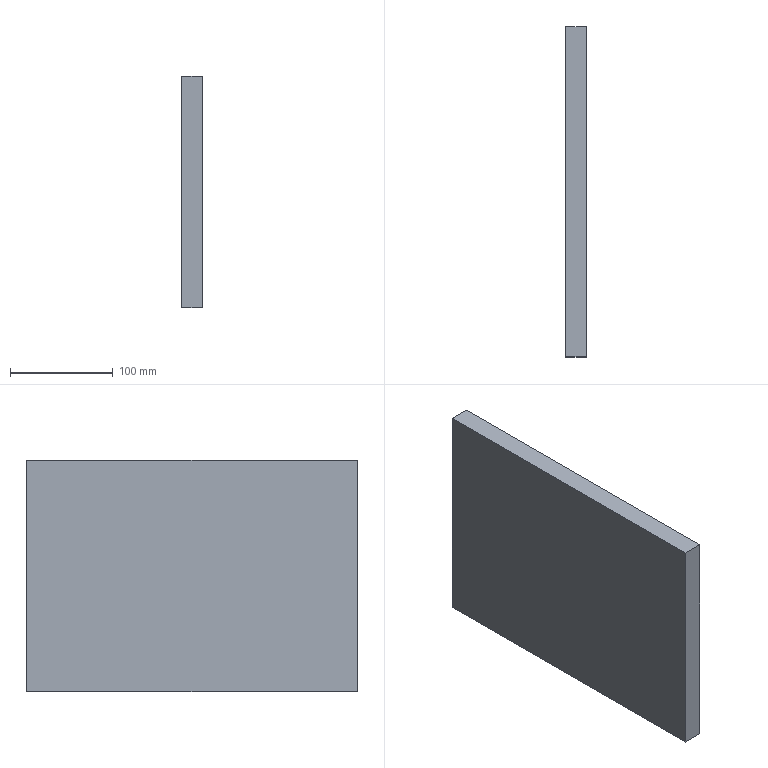Component | NX | CH3404_5-3 | 1 solid | 6 faces | box 20 x 321 x 225 mm | volume 1444500 mm3 | plane 6
STEP:
#1=CARTESIAN_POINT('',(0.,0.,0.));
#2=DIRECTION('',(0.,0.,1.));
#3=DIRECTION('',(1.,0.,0.));
#4=AXIS2_PLACEMENT_3D('',#1,#2,#3);
#5=CARTESIAN_POINT('',(115.,-160.5,0.));
#6=VERTEX_POINT('',#5);
#7=CARTESIAN_POINT('',(115.,160.5,-0.));
#8=VERTEX_POINT('',#7);
#9=CARTESIAN_POINT('',(115.,-160.5,0.));
#10=DIRECTION('',(0.,1.,-0.));
#11=VECTOR('',#10,1.);
#12=LINE('',#9,#11);
#13=CARTESIAN_POINT('',(95.,-160.5,0.));
#14=DIRECTION('',(0.,-0.,-1.));
#15=DIRECTION('',(0.,-1.,0.));
#16=AXIS2_PLACEMENT_3D('',#13,#14,#15);
#17=PLANE('',#16);
#18=CARTESIAN_POINT('',(0.,-20.));
#19=DIRECTION('',(-1.,0.));
#20=VECTOR('',#19,1.);
#21=LINE('',#18,#20);
#22=(GEOMETRIC_REPRESENTATION_CONTEXT(2)PARAMETRIC_REPRESENTATION_CONTEXT()REPRESENTATION_CONTEXT('',''));
#23=DEFINITIONAL_REPRESENTATION('',(#21),#22);
#24=PCURVE('',#17,#23);
#25=CARTESIAN_POINT('',(115.,160.5,-112.5));
#26=DIRECTION('',(-1.,0.,0.));
#27=DIRECTION('',(0.,1.,0.));
#28=AXIS2_PLACEMENT_3D('',#25,#26,#27);
#29=PLANE('',#28);
#30=CARTESIAN_POINT('',(-321.,-112.5));
#31=DIRECTION('',(1.,0.));
#32=VECTOR('',#31,1.);
#33=LINE('',#30,#32);
#34=(GEOMETRIC_REPRESENTATION_CONTEXT(2)PARAMETRIC_REPRESENTATION_CONTEXT()REPRESENTATION_CONTEXT('',''));
#35=DEFINITIONAL_REPRESENTATION('',(#33),#34);
#36=PCURVE('',#29,#35);
#37=SURFACE_CURVE('',#12,(#24,#36),.PCURVE_S1.);
#38=EDGE_CURVE('',#6,#8,#37,.T.);
#39=ORIENTED_EDGE('',*,*,#38,.T.);
#40=CARTESIAN_POINT('',(95.,160.5,-0.));
#41=VERTEX_POINT('',#40);
#42=CARTESIAN_POINT('',(95.,160.5,-0.));
#43=DIRECTION('',(1.,0.,0.));
#44=VECTOR('',#43,1.);
#45=LINE('',#42,#44);
#46=CARTESIAN_POINT('',(-321.,0.));
#47=DIRECTION('',(0.,-1.));
#48=VECTOR('',#47,1.);
#49=LINE('',#46,#48);
#50=(GEOMETRIC_REPRESENTATION_CONTEXT(2)PARAMETRIC_REPRESENTATION_CONTEXT()REPRESENTATION_CONTEXT('',''));
#51=DEFINITIONAL_REPRESENTATION('',(#49),#50);
#52=PCURVE('',#17,#51);
#53=CARTESIAN_POINT('',(95.,160.5,-0.));
#54=DIRECTION('',(0.,-1.,0.));
#55=DIRECTION('',(-1.,0.,0.));
#56=AXIS2_PLACEMENT_3D('',#53,#54,#55);
#57=PLANE('',#56);
#58=CARTESIAN_POINT('',(0.,0.));
#59=DIRECTION('',(-1.,0.));
#60=VECTOR('',#59,1.);
#61=LINE('',#58,#60);
#62=(GEOMETRIC_REPRESENTATION_CONTEXT(2)PARAMETRIC_REPRESENTATION_CONTEXT()REPRESENTATION_CONTEXT('',''));
#63=DEFINITIONAL_REPRESENTATION('',(#61),#62);
#64=PCURVE('',#57,#63);
#65=SURFACE_CURVE('',#45,(#52,#64),.PCURVE_S1.);
#66=EDGE_CURVE('',#41,#8,#65,.T.);
#67=ORIENTED_EDGE('',*,*,#66,.F.);
#68=CARTESIAN_POINT('',(95.,-160.5,0.));
#69=VERTEX_POINT('',#68);
#70=CARTESIAN_POINT('',(95.,-160.5,0.));
#71=DIRECTION('',(0.,1.,-0.));
#72=VECTOR('',#71,1.);
#73=LINE('',#70,#72);
#74=CARTESIAN_POINT('',(0.,0.));
#75=DIRECTION('',(-1.,0.));
#76=VECTOR('',#75,1.);
#77=LINE('',#74,#76);
#78=(GEOMETRIC_REPRESENTATION_CONTEXT(2)PARAMETRIC_REPRESENTATION_CONTEXT()REPRESENTATION_CONTEXT('',''));
#79=DEFINITIONAL_REPRESENTATION('',(#77),#78);
#80=PCURVE('',#17,#79);
#81=CARTESIAN_POINT('',(95.,160.5,-112.5));
#82=DIRECTION('',(-1.,0.,0.));
#83=DIRECTION('',(0.,1.,0.));
#84=AXIS2_PLACEMENT_3D('',#81,#82,#83);
#85=PLANE('',#84);
#86=CARTESIAN_POINT('',(-321.,-112.5));
#87=DIRECTION('',(1.,0.));
#88=VECTOR('',#87,1.);
#89=LINE('',#86,#88);
#90=(GEOMETRIC_REPRESENTATION_CONTEXT(2)PARAMETRIC_REPRESENTATION_CONTEXT()REPRESENTATION_CONTEXT('',''));
#91=DEFINITIONAL_REPRESENTATION('',(#89),#90);
#92=PCURVE('',#85,#91);
#93=SURFACE_CURVE('',#73,(#80,#92),.PCURVE_S1.);
#94=EDGE_CURVE('',#69,#41,#93,.T.);
#95=ORIENTED_EDGE('',*,*,#94,.F.);
#96=CARTESIAN_POINT('',(95.,-160.5,0.));
#97=DIRECTION('',(1.,0.,0.));
#98=VECTOR('',#97,1.);
#99=LINE('',#96,#98);
#100=CARTESIAN_POINT('',(0.,0.));
#101=DIRECTION('',(0.,-1.));
#102=VECTOR('',#101,1.);
#103=LINE('',#100,#102);
#104=(GEOMETRIC_REPRESENTATION_CONTEXT(2)PARAMETRIC_REPRESENTATION_CONTEXT()REPRESENTATION_CONTEXT('',''));
#105=DEFINITIONAL_REPRESENTATION('',(#103),#104);
#106=PCURVE('',#17,#105);
#107=CARTESIAN_POINT('',(95.,-160.5,-225.));
#108=DIRECTION('',(0.,1.,0.));
#109=DIRECTION('',(1.,0.,0.));
#110=AXIS2_PLACEMENT_3D('',#107,#108,#109);
#111=PLANE('',#110);
#112=CARTESIAN_POINT('',(0.,-225.));
#113=DIRECTION('',(1.,0.));
#114=VECTOR('',#113,1.);
#115=LINE('',#112,#114);
#116=(GEOMETRIC_REPRESENTATION_CONTEXT(2)PARAMETRIC_REPRESENTATION_CONTEXT()REPRESENTATION_CONTEXT('',''));
#117=DEFINITIONAL_REPRESENTATION('',(#115),#116);
#118=PCURVE('',#111,#117);
#119=SURFACE_CURVE('',#99,(#106,#118),.PCURVE_S1.);
#120=EDGE_CURVE('',#69,#6,#119,.T.);
#121=ORIENTED_EDGE('',*,*,#120,.T.);
#122=EDGE_LOOP('',(#39,#67,#95,#121));
#123=FACE_BOUND('',#122,.T.);
#124=ADVANCED_FACE('',(#123),#17,.F.);
#125=CARTESIAN_POINT('',(115.,160.5,-225.));
#126=VERTEX_POINT('',#125);
#127=CARTESIAN_POINT('',(115.,160.5,-0.));
#128=DIRECTION('',(0.,0.,-1.));
#129=VECTOR('',#128,1.);
#130=LINE('',#127,#129);
#131=CARTESIAN_POINT('',(-20.,0.));
#132=DIRECTION('',(0.,1.));
#133=VECTOR('',#132,1.);
#134=LINE('',#131,#133);
#135=(GEOMETRIC_REPRESENTATION_CONTEXT(2)PARAMETRIC_REPRESENTATION_CONTEXT()REPRESENTATION_CONTEXT('',''));
#136=DEFINITIONAL_REPRESENTATION('',(#134),#135);
#137=PCURVE('',#57,#136);
#138=CARTESIAN_POINT('',(0.,-112.5));
#139=DIRECTION('',(0.,1.));
#140=VECTOR('',#139,1.);
#141=LINE('',#138,#140);
#142=(GEOMETRIC_REPRESENTATION_CONTEXT(2)PARAMETRIC_REPRESENTATION_CONTEXT()REPRESENTATION_CONTEXT('',''));
#143=DEFINITIONAL_REPRESENTATION('',(#141),#142);
#144=PCURVE('',#29,#143);
#145=SURFACE_CURVE('',#130,(#137,#144),.PCURVE_S1.);
#146=EDGE_CURVE('',#8,#126,#145,.T.);
#147=ORIENTED_EDGE('',*,*,#146,.T.);
#148=CARTESIAN_POINT('',(95.,160.5,-225.));
#149=VERTEX_POINT('',#148);
#150=CARTESIAN_POINT('',(95.,160.5,-225.));
#151=DIRECTION('',(1.,0.,0.));
#152=VECTOR('',#151,1.);
#153=LINE('',#150,#152);
#154=CARTESIAN_POINT('',(0.,225.));
#155=DIRECTION('',(-1.,0.));
#156=VECTOR('',#155,1.);
#157=LINE('',#154,#156);
#158=(GEOMETRIC_REPRESENTATION_CONTEXT(2)PARAMETRIC_REPRESENTATION_CONTEXT()REPRESENTATION_CONTEXT('',''));
#159=DEFINITIONAL_REPRESENTATION('',(#157),#158);
#160=PCURVE('',#57,#159);
#161=CARTESIAN_POINT('',(95.,160.5,-225.));
#162=DIRECTION('',(0.,-0.,1.));
#163=DIRECTION('',(0.,1.,0.));
#164=AXIS2_PLACEMENT_3D('',#161,#162,#163);
#165=PLANE('',#164);
#166=CARTESIAN_POINT('',(0.,0.));
#167=DIRECTION('',(0.,-1.));
#168=VECTOR('',#167,1.);
#169=LINE('',#166,#168);
#170=(GEOMETRIC_REPRESENTATION_CONTEXT(2)PARAMETRIC_REPRESENTATION_CONTEXT()REPRESENTATION_CONTEXT('',''));
#171=DEFINITIONAL_REPRESENTATION('',(#169),#170);
#172=PCURVE('',#165,#171);
#173=SURFACE_CURVE('',#153,(#160,#172),.PCURVE_S1.);
#174=EDGE_CURVE('',#149,#126,#173,.T.);
#175=ORIENTED_EDGE('',*,*,#174,.F.);
#176=CARTESIAN_POINT('',(95.,160.5,-0.));
#177=DIRECTION('',(0.,0.,-1.));
#178=VECTOR('',#177,1.);
#179=LINE('',#176,#178);
#180=CARTESIAN_POINT('',(0.,0.));
#181=DIRECTION('',(0.,1.));
#182=VECTOR('',#181,1.);
#183=LINE('',#180,#182);
#184=(GEOMETRIC_REPRESENTATION_CONTEXT(2)PARAMETRIC_REPRESENTATION_CONTEXT()REPRESENTATION_CONTEXT('',''));
#185=DEFINITIONAL_REPRESENTATION('',(#183),#184);
#186=PCURVE('',#57,#185);
#187=CARTESIAN_POINT('',(0.,-112.5));
#188=DIRECTION('',(0.,1.));
#189=VECTOR('',#188,1.);
#190=LINE('',#187,#189);
#191=(GEOMETRIC_REPRESENTATION_CONTEXT(2)PARAMETRIC_REPRESENTATION_CONTEXT()REPRESENTATION_CONTEXT('',''));
#192=DEFINITIONAL_REPRESENTATION('',(#190),#191);
#193=PCURVE('',#85,#192);
#194=SURFACE_CURVE('',#179,(#186,#193),.PCURVE_S1.);
#195=EDGE_CURVE('',#41,#149,#194,.T.);
#196=ORIENTED_EDGE('',*,*,#195,.F.);
#197=ORIENTED_EDGE('',*,*,#66,.T.);
#198=EDGE_LOOP('',(#147,#175,#196,#197));
#199=FACE_BOUND('',#198,.T.);
#200=ADVANCED_FACE('',(#199),#57,.F.);
#201=CARTESIAN_POINT('',(115.,-160.5,-225.));
#202=VERTEX_POINT('',#201);
#203=CARTESIAN_POINT('',(115.,160.5,-225.));
#204=DIRECTION('',(0.,-1.,-0.));
#205=VECTOR('',#204,1.);
#206=LINE('',#203,#205);
#207=CARTESIAN_POINT('',(0.,-20.));
#208=DIRECTION('',(-1.,0.));
#209=VECTOR('',#208,1.);
#210=LINE('',#207,#209);
#211=(GEOMETRIC_REPRESENTATION_CONTEXT(2)PARAMETRIC_REPRESENTATION_CONTEXT()REPRESENTATION_CONTEXT('',''));
#212=DEFINITIONAL_REPRESENTATION('',(#210),#211);
#213=PCURVE('',#165,#212);
#214=CARTESIAN_POINT('',(0.,112.5));
#215=DIRECTION('',(-1.,0.));
#216=VECTOR('',#215,1.);
#217=LINE('',#214,#216);
#218=(GEOMETRIC_REPRESENTATION_CONTEXT(2)PARAMETRIC_REPRESENTATION_CONTEXT()REPRESENTATION_CONTEXT('',''));
#219=DEFINITIONAL_REPRESENTATION('',(#217),#218);
#220=PCURVE('',#29,#219);
#221=SURFACE_CURVE('',#206,(#213,#220),.PCURVE_S1.);
#222=EDGE_CURVE('',#126,#202,#221,.T.);
#223=ORIENTED_EDGE('',*,*,#222,.T.);
#224=CARTESIAN_POINT('',(95.,-160.5,-225.));
#225=VERTEX_POINT('',#224);
#226=CARTESIAN_POINT('',(95.,-160.5,-225.));
#227=DIRECTION('',(1.,0.,0.));
#228=VECTOR('',#227,1.);
#229=LINE('',#226,#228);
#230=CARTESIAN_POINT('',(-321.,0.));
#231=DIRECTION('',(0.,-1.));
#232=VECTOR('',#231,1.);
#233=LINE('',#230,#232);
#234=(GEOMETRIC_REPRESENTATION_CONTEXT(2)PARAMETRIC_REPRESENTATION_CONTEXT()REPRESENTATION_CONTEXT('',''));
#235=DEFINITIONAL_REPRESENTATION('',(#233),#234);
#236=PCURVE('',#165,#235);
#237=CARTESIAN_POINT('',(0.,0.));
#238=DIRECTION('',(1.,0.));
#239=VECTOR('',#238,1.);
#240=LINE('',#237,#239);
#241=(GEOMETRIC_REPRESENTATION_CONTEXT(2)PARAMETRIC_REPRESENTATION_CONTEXT()REPRESENTATION_CONTEXT('',''));
#242=DEFINITIONAL_REPRESENTATION('',(#240),#241);
#243=PCURVE('',#111,#242);
#244=SURFACE_CURVE('',#229,(#236,#243),.PCURVE_S1.);
#245=EDGE_CURVE('',#225,#202,#244,.T.);
#246=ORIENTED_EDGE('',*,*,#245,.F.);
#247=CARTESIAN_POINT('',(95.,160.5,-225.));
#248=DIRECTION('',(0.,-1.,-0.));
#249=VECTOR('',#248,1.);
#250=LINE('',#247,#249);
#251=CARTESIAN_POINT('',(0.,0.));
#252=DIRECTION('',(-1.,0.));
#253=VECTOR('',#252,1.);
#254=LINE('',#251,#253);
#255=(GEOMETRIC_REPRESENTATION_CONTEXT(2)PARAMETRIC_REPRESENTATION_CONTEXT()REPRESENTATION_CONTEXT('',''));
#256=DEFINITIONAL_REPRESENTATION('',(#254),#255);
#257=PCURVE('',#165,#256);
#258=CARTESIAN_POINT('',(0.,112.5));
#259=DIRECTION('',(-1.,0.));
#260=VECTOR('',#259,1.);
#261=LINE('',#258,#260);
#262=(GEOMETRIC_REPRESENTATION_CONTEXT(2)PARAMETRIC_REPRESENTATION_CONTEXT()REPRESENTATION_CONTEXT('',''));
#263=DEFINITIONAL_REPRESENTATION('',(#261),#262);
#264=PCURVE('',#85,#263);
#265=SURFACE_CURVE('',#250,(#257,#264),.PCURVE_S1.);
#266=EDGE_CURVE('',#149,#225,#265,.T.);
#267=ORIENTED_EDGE('',*,*,#266,.F.);
#268=ORIENTED_EDGE('',*,*,#174,.T.);
#269=EDGE_LOOP('',(#223,#246,#267,#268));
#270=FACE_BOUND('',#269,.T.);
#271=ADVANCED_FACE('',(#270),#165,.F.);
#272=CARTESIAN_POINT('',(115.,-160.5,-225.));
#273=DIRECTION('',(0.,0.,1.));
#274=VECTOR('',#273,1.);
#275=LINE('',#272,#274);
#276=CARTESIAN_POINT('',(20.,0.));
#277=DIRECTION('',(0.,-1.));
#278=VECTOR('',#277,1.);
#279=LINE('',#276,#278);
#280=(GEOMETRIC_REPRESENTATION_CONTEXT(2)PARAMETRIC_REPRESENTATION_CONTEXT()REPRESENTATION_CONTEXT('',''));
#281=DEFINITIONAL_REPRESENTATION('',(#279),#280);
#282=PCURVE('',#111,#281);
#283=CARTESIAN_POINT('',(-321.,112.5));
#284=DIRECTION('',(0.,-1.));
#285=VECTOR('',#284,1.);
#286=LINE('',#283,#285);
#287=(GEOMETRIC_REPRESENTATION_CONTEXT(2)PARAMETRIC_REPRESENTATION_CONTEXT()REPRESENTATION_CONTEXT('',''));
#288=DEFINITIONAL_REPRESENTATION('',(#286),#287);
#289=PCURVE('',#29,#288);
#290=SURFACE_CURVE('',#275,(#282,#289),.PCURVE_S1.);
#291=EDGE_CURVE('',#202,#6,#290,.T.);
#292=ORIENTED_EDGE('',*,*,#291,.T.);
#293=ORIENTED_EDGE('',*,*,#120,.F.);
#294=CARTESIAN_POINT('',(95.,-160.5,-225.));
#295=DIRECTION('',(0.,0.,1.));
#296=VECTOR('',#295,1.);
#297=LINE('',#294,#296);
#298=CARTESIAN_POINT('',(0.,0.));
#299=DIRECTION('',(0.,-1.));
#300=VECTOR('',#299,1.);
#301=LINE('',#298,#300);
#302=(GEOMETRIC_REPRESENTATION_CONTEXT(2)PARAMETRIC_REPRESENTATION_CONTEXT()REPRESENTATION_CONTEXT('',''));
#303=DEFINITIONAL_REPRESENTATION('',(#301),#302);
#304=PCURVE('',#111,#303);
#305=CARTESIAN_POINT('',(-321.,112.5));
#306=DIRECTION('',(0.,-1.));
#307=VECTOR('',#306,1.);
#308=LINE('',#305,#307);
#309=(GEOMETRIC_REPRESENTATION_CONTEXT(2)PARAMETRIC_REPRESENTATION_CONTEXT()REPRESENTATION_CONTEXT('',''));
#310=DEFINITIONAL_REPRESENTATION('',(#308),#309);
#311=PCURVE('',#85,#310);
#312=SURFACE_CURVE('',#297,(#304,#311),.PCURVE_S1.);
#313=EDGE_CURVE('',#225,#69,#312,.T.);
#314=ORIENTED_EDGE('',*,*,#313,.F.);
#315=ORIENTED_EDGE('',*,*,#245,.T.);
#316=EDGE_LOOP('',(#292,#293,#314,#315));
#317=FACE_BOUND('',#316,.T.);
#318=ADVANCED_FACE('',(#317),#111,.F.);
#319=ORIENTED_EDGE('',*,*,#94,.T.);
#320=ORIENTED_EDGE('',*,*,#195,.T.);
#321=ORIENTED_EDGE('',*,*,#266,.T.);
#322=ORIENTED_EDGE('',*,*,#313,.T.);
#323=EDGE_LOOP('',(#319,#320,#321,#322));
#324=FACE_BOUND('',#323,.T.);
#325=ADVANCED_FACE('',(#324),#85,.T.);
#326=ORIENTED_EDGE('',*,*,#38,.F.);
#327=ORIENTED_EDGE('',*,*,#291,.F.);
#328=ORIENTED_EDGE('',*,*,#222,.F.);
#329=ORIENTED_EDGE('',*,*,#146,.F.);
#330=EDGE_LOOP('',(#326,#327,#328,#329));
#331=FACE_BOUND('',#330,.T.);
#332=ADVANCED_FACE('',(#331),#29,.F.);
#333=CLOSED_SHELL('',(#124,#200,#271,#318,#325,#332));
#334=MANIFOLD_SOLID_BREP('',#333);
#335=(LENGTH_UNIT()NAMED_UNIT(*)SI_UNIT(.MILLI.,.METRE.));
#336=UNCERTAINTY_MEASURE_WITH_UNIT(LENGTH_MEASURE(0.0000001),#335,'','');
#337=(NAMED_UNIT(*)PLANE_ANGLE_UNIT()SI_UNIT($,.RADIAN.));
#338=(NAMED_UNIT(*)SI_UNIT($,.STERADIAN.)SOLID_ANGLE_UNIT());
#339=(GEOMETRIC_REPRESENTATION_CONTEXT(3)GLOBAL_UNCERTAINTY_ASSIGNED_CONTEXT((#336))GLOBAL_UNIT_ASSIGNED_CONTEXT((#335,#337,#338))REPRESENTATION_CONTEXT('',''));
#340=ADVANCED_BREP_SHAPE_REPRESENTATION('',(#4,#334),#339);